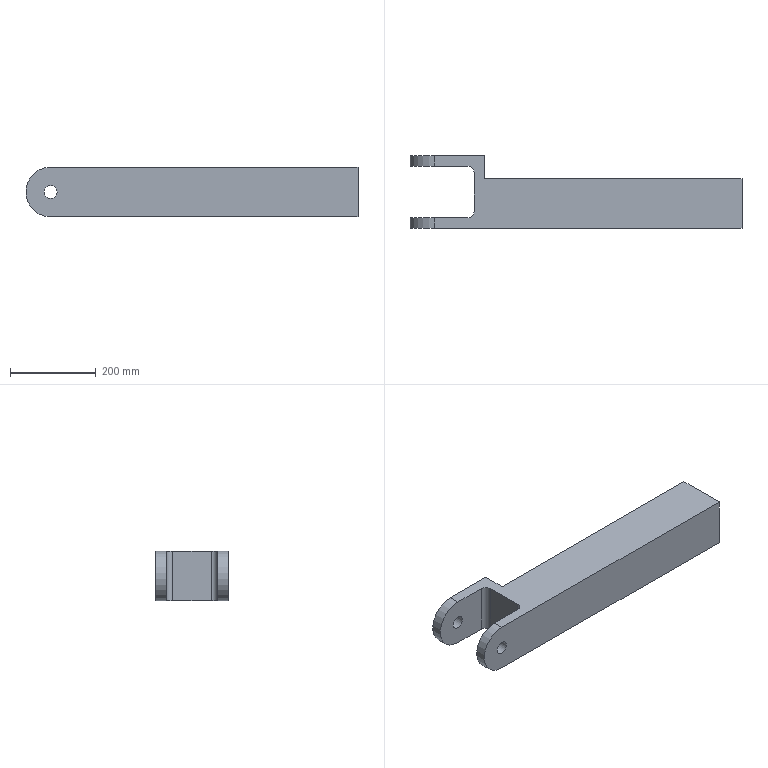Component | NX | SWING_ROD | 1 solid | 21 faces | volume 3810667 mm3 | plane 15 | cylinder 6 | commonest cylinder face diameters 30 x4 116 x2